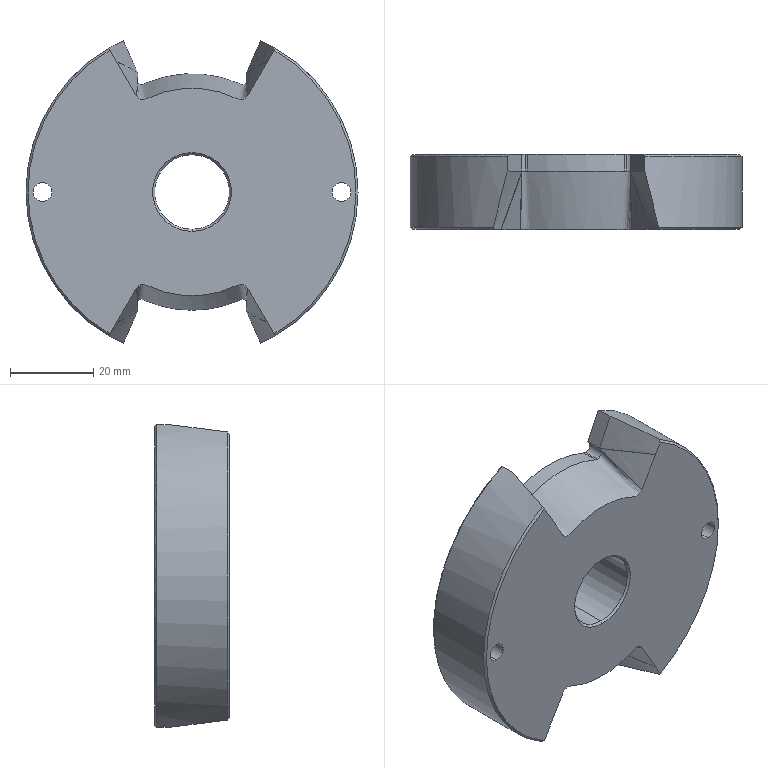Component | SolidWorks | 5-1 | 1 solid | 63 faces | volume 68659 mm3 | cylinder 31 | spline 14 | plane 10 | cone 8 | commonest cylinder face diameters 3 x6 6 x6 4.5 x4 57 x3 29 x2 37 x2 18 x2 80 x2